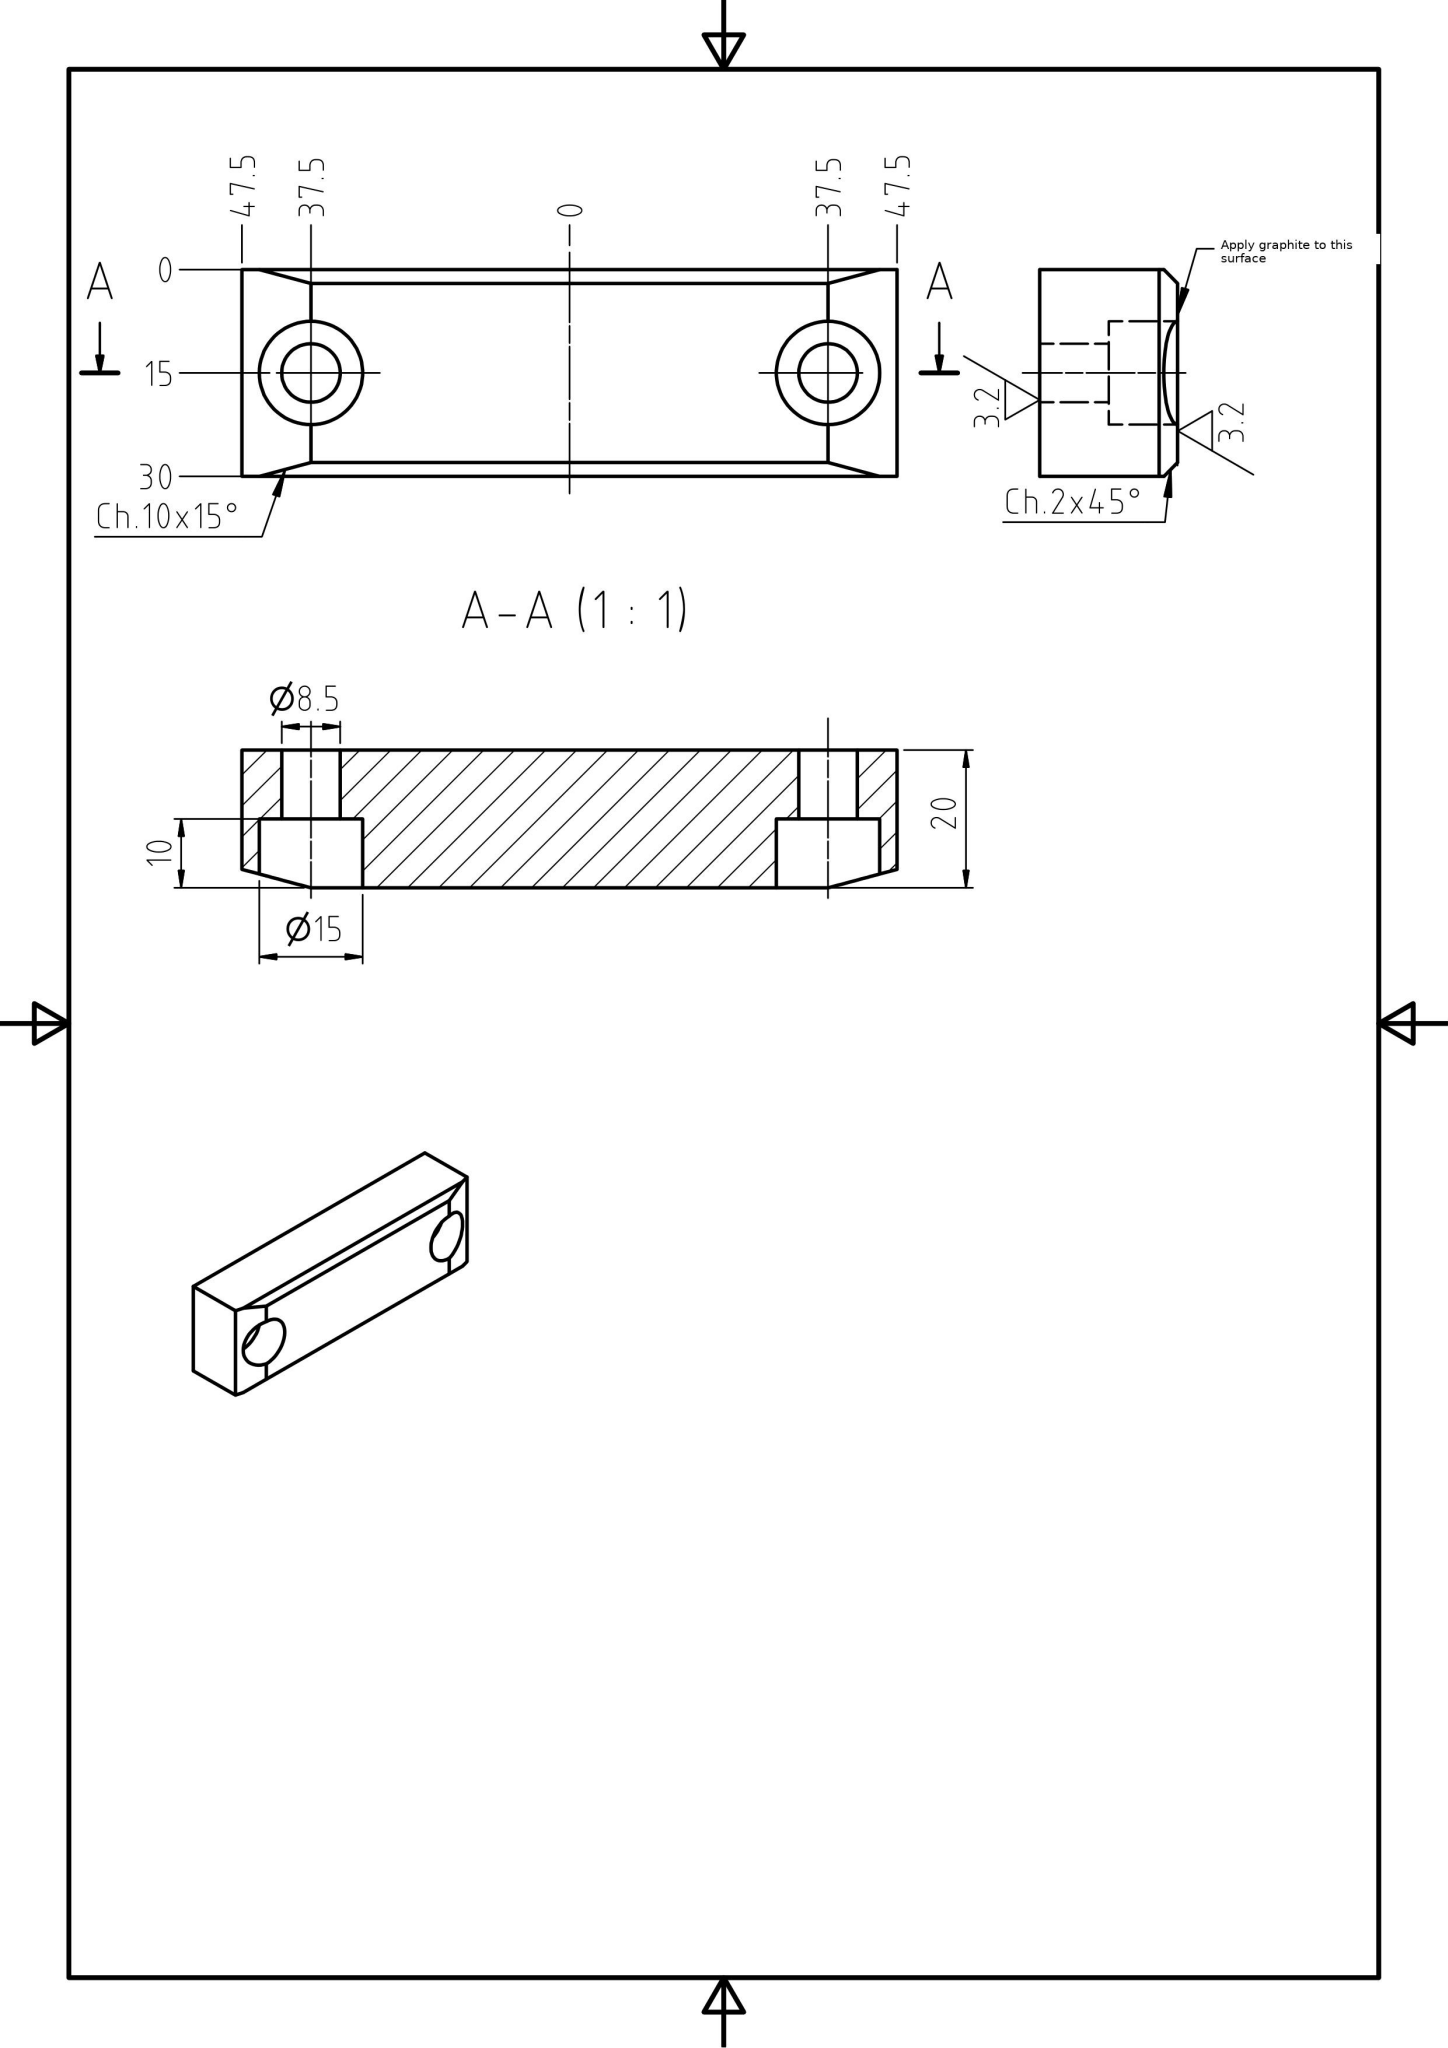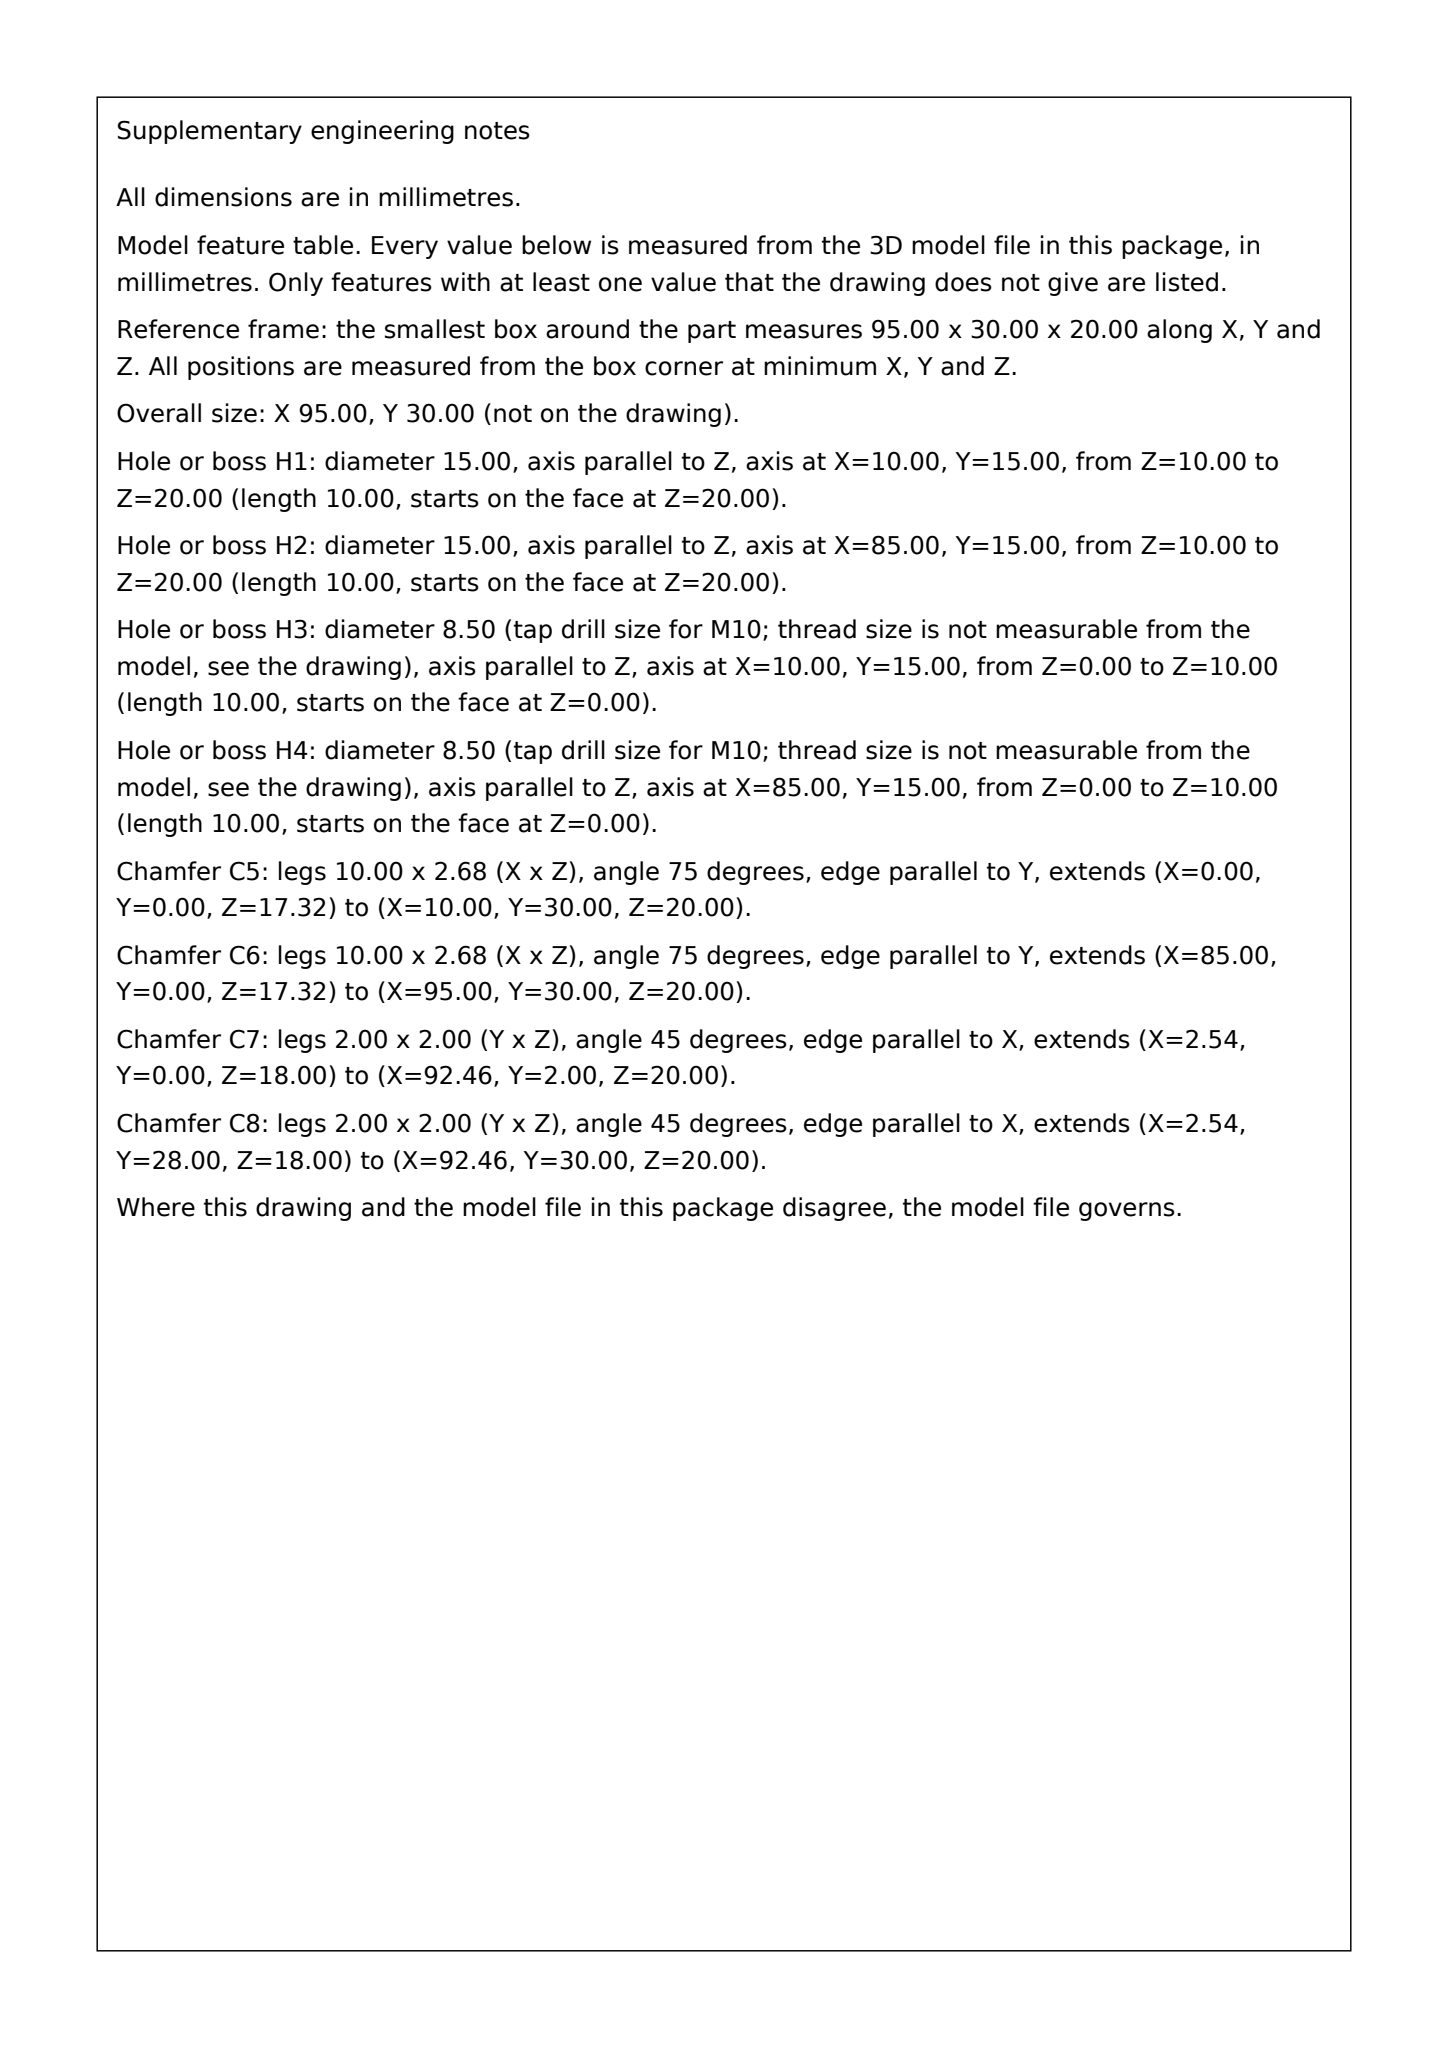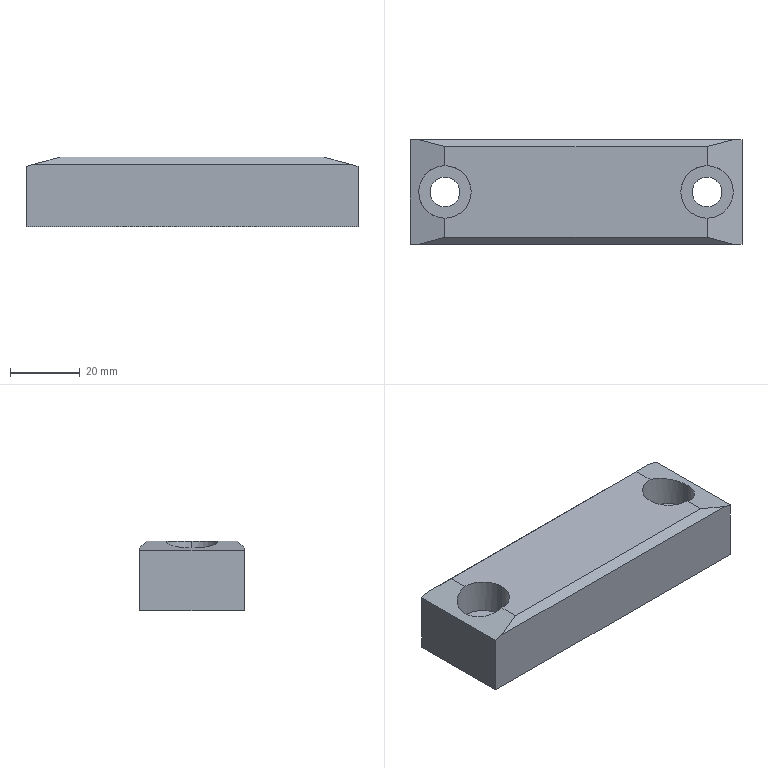Part | SolidWorks | mm | 1 solid | 20 faces | box 95 x 30 x 20 mm | volume 51358 mm3 | plane 12 | cylinder 8 | commonest cylinder face diameters 8.5 x4 15 x4
STEP:
#1=CARTESIAN_POINT('',(33.25,0.,0.));
#2=VERTEX_POINT('',#1);
#3=CARTESIAN_POINT('',(41.75,0.,0.));
#4=VERTEX_POINT('',#3);
#5=CARTESIAN_POINT('',(37.5,0.,0.));
#6=DIRECTION('',(0.,0.,1.));
#7=DIRECTION('',(1.,0.,0.));
#8=AXIS2_PLACEMENT_3D('',#5,#6,#7);
#9=CIRCLE('',#8,4.25);
#10=EDGE_CURVE('',#2,#4,#9,.T.);
#11=ORIENTED_EDGE('',*,*,#10,.F.);
#12=CARTESIAN_POINT('',(33.25,0.,10.));
#13=VERTEX_POINT('',#12);
#14=CARTESIAN_POINT('',(33.25,0.,5.));
#15=DIRECTION('',(0.,0.,1.));
#16=VECTOR('',#15,1000.);
#17=LINE('',#14,#16);
#18=EDGE_CURVE('',#2,#13,#17,.T.);
#19=ORIENTED_EDGE('',*,*,#18,.T.);
#20=CARTESIAN_POINT('',(41.75,0.,10.));
#21=VERTEX_POINT('',#20);
#22=CARTESIAN_POINT('',(37.5,0.,10.));
#23=DIRECTION('',(0.,0.,1.));
#24=DIRECTION('',(1.,0.,0.));
#25=AXIS2_PLACEMENT_3D('',#22,#23,#24);
#26=CIRCLE('',#25,4.25);
#27=EDGE_CURVE('',#13,#21,#26,.T.);
#28=ORIENTED_EDGE('',*,*,#27,.T.);
#29=CARTESIAN_POINT('',(41.75,0.,5.));
#30=DIRECTION('',(0.,0.,1.));
#31=VECTOR('',#30,1000.);
#32=LINE('',#29,#31);
#33=EDGE_CURVE('',#4,#21,#32,.T.);
#34=ORIENTED_EDGE('',*,*,#33,.F.);
#35=EDGE_LOOP('',(#11,#19,#28,#34));
#36=FACE_OUTER_BOUND('',#35,.T.);
#37=CARTESIAN_POINT('',(37.5,0.,5.));
#38=DIRECTION('',(0.,0.,1.));
#39=DIRECTION('',(1.,0.,0.));
#40=AXIS2_PLACEMENT_3D('',#37,#38,#39);
#41=CYLINDRICAL_SURFACE('',#40,4.25);
#42=ADVANCED_FACE('',(#36),#41,.F.);
#43=CARTESIAN_POINT('',(30.,0.,10.));
#44=VERTEX_POINT('',#43);
#45=CARTESIAN_POINT('',(45.,0.,10.));
#46=VERTEX_POINT('',#45);
#47=CARTESIAN_POINT('',(37.5,0.,10.));
#48=DIRECTION('',(0.,0.,1.));
#49=DIRECTION('',(1.,0.,0.));
#50=AXIS2_PLACEMENT_3D('',#47,#48,#49);
#51=CIRCLE('',#50,7.5);
#52=EDGE_CURVE('',#44,#46,#51,.T.);
#53=ORIENTED_EDGE('',*,*,#52,.F.);
#54=CARTESIAN_POINT('',(30.,0.,20.));
#55=VERTEX_POINT('',#54);
#56=CARTESIAN_POINT('',(30.,0.,15.));
#57=DIRECTION('',(0.,0.,1.));
#58=VECTOR('',#57,1000.);
#59=LINE('',#56,#58);
#60=EDGE_CURVE('',#44,#55,#59,.T.);
#61=ORIENTED_EDGE('',*,*,#60,.T.);
#62=CARTESIAN_POINT('',(37.5,-7.5,20.));
#63=VERTEX_POINT('',#62);
#64=CARTESIAN_POINT('',(37.5,0.,20.));
#65=DIRECTION('',(0.,0.,-1.));
#66=DIRECTION('',(1.,0.,0.));
#67=AXIS2_PLACEMENT_3D('',#64,#65,#66);
#68=CIRCLE('',#67,7.5);
#69=EDGE_CURVE('',#63,#55,#68,.T.);
#70=ORIENTED_EDGE('',*,*,#69,.F.);
#71=CARTESIAN_POINT('',(45.,0.,17.99));
#72=VERTEX_POINT('',#71);
#73=CARTESIAN_POINT('',(45.,0.,17.99));
#74=CARTESIAN_POINT('',(45.,-4.393,17.99));
#75=CARTESIAN_POINT('',(41.893,-7.5,18.823));
#76=CARTESIAN_POINT('',(37.5,-7.5,20.));
#77=(BOUNDED_CURVE()B_SPLINE_CURVE(3,(#73,#74,#75,#76),.UNSPECIFIED.,.F.,.F.)B_SPLINE_CURVE_WITH_KNOTS((4,4),(0.,1.571),.UNSPECIFIED.)CURVE()GEOMETRIC_REPRESENTATION_ITEM()RATIONAL_B_SPLINE_CURVE((1.,0.8047,0.8047,1.))REPRESENTATION_ITEM(''));
#78=EDGE_CURVE('',#72,#63,#77,.T.);
#79=ORIENTED_EDGE('',*,*,#78,.F.);
#80=CARTESIAN_POINT('',(45.,0.,15.));
#81=DIRECTION('',(0.,0.,1.));
#82=VECTOR('',#81,1000.);
#83=LINE('',#80,#82);
#84=EDGE_CURVE('',#46,#72,#83,.T.);
#85=ORIENTED_EDGE('',*,*,#84,.F.);
#86=EDGE_LOOP('',(#53,#61,#70,#79,#85));
#87=FACE_OUTER_BOUND('',#86,.T.);
#88=CARTESIAN_POINT('',(37.5,0.,15.));
#89=DIRECTION('',(0.,0.,1.));
#90=DIRECTION('',(1.,0.,0.));
#91=AXIS2_PLACEMENT_3D('',#88,#89,#90);
#92=CYLINDRICAL_SURFACE('',#91,7.5);
#93=ADVANCED_FACE('',(#87),#92,.F.);
#94=CARTESIAN_POINT('',(-41.75,0.,0.));
#95=VERTEX_POINT('',#94);
#96=CARTESIAN_POINT('',(-33.25,0.,0.));
#97=VERTEX_POINT('',#96);
#98=CARTESIAN_POINT('',(-37.5,0.,0.));
#99=DIRECTION('',(0.,0.,1.));
#100=DIRECTION('',(1.,0.,0.));
#101=AXIS2_PLACEMENT_3D('',#98,#99,#100);
#102=CIRCLE('',#101,4.25);
#103=EDGE_CURVE('',#95,#97,#102,.T.);
#104=ORIENTED_EDGE('',*,*,#103,.F.);
#105=CARTESIAN_POINT('',(-41.75,0.,10.));
#106=VERTEX_POINT('',#105);
#107=CARTESIAN_POINT('',(-41.75,0.,5.));
#108=DIRECTION('',(0.,0.,1.));
#109=VECTOR('',#108,1000.);
#110=LINE('',#107,#109);
#111=EDGE_CURVE('',#95,#106,#110,.T.);
#112=ORIENTED_EDGE('',*,*,#111,.T.);
#113=CARTESIAN_POINT('',(-33.25,0.,10.));
#114=VERTEX_POINT('',#113);
#115=CARTESIAN_POINT('',(-37.5,0.,10.));
#116=DIRECTION('',(0.,0.,1.));
#117=DIRECTION('',(1.,0.,0.));
#118=AXIS2_PLACEMENT_3D('',#115,#116,#117);
#119=CIRCLE('',#118,4.25);
#120=EDGE_CURVE('',#106,#114,#119,.T.);
#121=ORIENTED_EDGE('',*,*,#120,.T.);
#122=CARTESIAN_POINT('',(-33.25,0.,5.));
#123=DIRECTION('',(0.,0.,1.));
#124=VECTOR('',#123,1000.);
#125=LINE('',#122,#124);
#126=EDGE_CURVE('',#97,#114,#125,.T.);
#127=ORIENTED_EDGE('',*,*,#126,.F.);
#128=EDGE_LOOP('',(#104,#112,#121,#127));
#129=FACE_OUTER_BOUND('',#128,.T.);
#130=CARTESIAN_POINT('',(-37.5,0.,5.));
#131=DIRECTION('',(0.,0.,1.));
#132=DIRECTION('',(1.,0.,0.));
#133=AXIS2_PLACEMENT_3D('',#130,#131,#132);
#134=CYLINDRICAL_SURFACE('',#133,4.25);
#135=ADVANCED_FACE('',(#129),#134,.F.);
#136=CARTESIAN_POINT('',(-45.,0.,10.));
#137=VERTEX_POINT('',#136);
#138=CARTESIAN_POINT('',(-30.,0.,10.));
#139=VERTEX_POINT('',#138);
#140=CARTESIAN_POINT('',(-37.5,0.,10.));
#141=DIRECTION('',(0.,0.,1.));
#142=DIRECTION('',(1.,0.,0.));
#143=AXIS2_PLACEMENT_3D('',#140,#141,#142);
#144=CIRCLE('',#143,7.5);
#145=EDGE_CURVE('',#137,#139,#144,.T.);
#146=ORIENTED_EDGE('',*,*,#145,.F.);
#147=CARTESIAN_POINT('',(-45.,0.,17.99));
#148=VERTEX_POINT('',#147);
#149=CARTESIAN_POINT('',(-45.,0.,15.));
#150=DIRECTION('',(0.,0.,1.));
#151=VECTOR('',#150,1000.);
#152=LINE('',#149,#151);
#153=EDGE_CURVE('',#137,#148,#152,.T.);
#154=ORIENTED_EDGE('',*,*,#153,.T.);
#155=CARTESIAN_POINT('',(-37.5,-7.5,20.));
#156=VERTEX_POINT('',#155);
#157=CARTESIAN_POINT('',(-37.5,-7.5,20.));
#158=CARTESIAN_POINT('',(-41.893,-7.5,18.823));
#159=CARTESIAN_POINT('',(-45.,-4.393,17.99));
#160=CARTESIAN_POINT('',(-45.,0.,17.99));
#161=(BOUNDED_CURVE()B_SPLINE_CURVE(3,(#157,#158,#159,#160),.UNSPECIFIED.,.F.,.F.)B_SPLINE_CURVE_WITH_KNOTS((4,4),(1.571,3.142),.UNSPECIFIED.)CURVE()GEOMETRIC_REPRESENTATION_ITEM()RATIONAL_B_SPLINE_CURVE((1.,0.8047,0.8047,1.))REPRESENTATION_ITEM(''));
#162=EDGE_CURVE('',#156,#148,#161,.T.);
#163=ORIENTED_EDGE('',*,*,#162,.F.);
#164=CARTESIAN_POINT('',(-30.,0.,20.));
#165=VERTEX_POINT('',#164);
#166=CARTESIAN_POINT('',(-37.5,0.,20.));
#167=DIRECTION('',(0.,0.,-1.));
#168=DIRECTION('',(1.,0.,0.));
#169=AXIS2_PLACEMENT_3D('',#166,#167,#168);
#170=CIRCLE('',#169,7.5);
#171=EDGE_CURVE('',#165,#156,#170,.T.);
#172=ORIENTED_EDGE('',*,*,#171,.F.);
#173=CARTESIAN_POINT('',(-30.,0.,15.));
#174=DIRECTION('',(0.,0.,1.));
#175=VECTOR('',#174,1000.);
#176=LINE('',#173,#175);
#177=EDGE_CURVE('',#139,#165,#176,.T.);
#178=ORIENTED_EDGE('',*,*,#177,.F.);
#179=EDGE_LOOP('',(#146,#154,#163,#172,#178));
#180=FACE_OUTER_BOUND('',#179,.T.);
#181=CARTESIAN_POINT('',(-37.5,0.,15.));
#182=DIRECTION('',(0.,0.,1.));
#183=DIRECTION('',(1.,0.,0.));
#184=AXIS2_PLACEMENT_3D('',#181,#182,#183);
#185=CYLINDRICAL_SURFACE('',#184,7.5);
#186=ADVANCED_FACE('',(#180),#185,.F.);
#187=CARTESIAN_POINT('',(44.964,-15.,18.));
#188=VERTEX_POINT('',#187);
#189=CARTESIAN_POINT('',(37.5,-13.,20.));
#190=VERTEX_POINT('',#189);
#191=CARTESIAN_POINT('',(12.653,-6.342,26.658));
#192=DIRECTION('',(-0.9351,0.2506,0.2506));
#193=VECTOR('',#192,1000.);
#194=LINE('',#191,#193);
#195=EDGE_CURVE('',#188,#190,#194,.T.);
#196=ORIENTED_EDGE('',*,*,#195,.T.);
#197=CARTESIAN_POINT('',(-37.5,-13.,20.));
#198=VERTEX_POINT('',#197);
#199=CARTESIAN_POINT('',(-23.75,-13.,20.));
#200=DIRECTION('',(-1.,0.,0.));
#201=VECTOR('',#200,1000.);
#202=LINE('',#199,#201);
#203=EDGE_CURVE('',#190,#198,#202,.T.);
#204=ORIENTED_EDGE('',*,*,#203,.T.);
#205=CARTESIAN_POINT('',(-44.964,-15.,18.));
#206=VERTEX_POINT('',#205);
#207=CARTESIAN_POINT('',(-31.664,-11.436,21.564));
#208=DIRECTION('',(-0.9351,-0.2506,-0.2506));
#209=VECTOR('',#208,1000.);
#210=LINE('',#207,#209);
#211=EDGE_CURVE('',#198,#206,#210,.T.);
#212=ORIENTED_EDGE('',*,*,#211,.T.);
#213=CARTESIAN_POINT('',(-23.75,-15.,18.));
#214=DIRECTION('',(1.,0.,0.));
#215=VECTOR('',#214,1000.);
#216=LINE('',#213,#215);
#217=EDGE_CURVE('',#206,#188,#216,.T.);
#218=ORIENTED_EDGE('',*,*,#217,.T.);
#219=EDGE_LOOP('',(#196,#204,#212,#218));
#220=FACE_OUTER_BOUND('',#219,.T.);
#221=CARTESIAN_POINT('',(-23.75,-14.,19.));
#222=DIRECTION('',(0.,-0.7071,0.7071));
#223=DIRECTION('',(-1.,0.,0.));
#224=AXIS2_PLACEMENT_3D('',#221,#222,#223);
#225=PLANE('',#224);
#226=ADVANCED_FACE('',(#220),#225,.T.);
#227=ORIENTED_EDGE('',*,*,#211,.F.);
#228=CARTESIAN_POINT('',(-37.5,7.5,20.));
#229=DIRECTION('',(0.,1.,0.));
#230=VECTOR('',#229,1000.);
#231=LINE('',#228,#230);
#232=EDGE_CURVE('',#198,#156,#231,.T.);
#233=ORIENTED_EDGE('',*,*,#232,.T.);
#234=ORIENTED_EDGE('',*,*,#162,.T.);
#235=CARTESIAN_POINT('',(-37.5,7.5,20.));
#236=VERTEX_POINT('',#235);
#237=CARTESIAN_POINT('',(-45.,0.,17.99));
#238=CARTESIAN_POINT('',(-45.,4.393,17.99));
#239=CARTESIAN_POINT('',(-41.893,7.5,18.823));
#240=CARTESIAN_POINT('',(-37.5,7.5,20.));
#241=(BOUNDED_CURVE()B_SPLINE_CURVE(3,(#237,#238,#239,#240),.UNSPECIFIED.,.F.,.F.)B_SPLINE_CURVE_WITH_KNOTS((4,4),(3.142,4.712),.UNSPECIFIED.)CURVE()GEOMETRIC_REPRESENTATION_ITEM()RATIONAL_B_SPLINE_CURVE((1.,0.8047,0.8047,1.))REPRESENTATION_ITEM(''));
#242=EDGE_CURVE('',#148,#236,#241,.T.);
#243=ORIENTED_EDGE('',*,*,#242,.T.);
#244=CARTESIAN_POINT('',(-37.5,13.,20.));
#245=VERTEX_POINT('',#244);
#246=CARTESIAN_POINT('',(-37.5,7.5,20.));
#247=DIRECTION('',(0.,1.,0.));
#248=VECTOR('',#247,1000.);
#249=LINE('',#246,#248);
#250=EDGE_CURVE('',#236,#245,#249,.T.);
#251=ORIENTED_EDGE('',*,*,#250,.T.);
#252=CARTESIAN_POINT('',(-44.964,15.,18.));
#253=VERTEX_POINT('',#252);
#254=CARTESIAN_POINT('',(-12.653,6.342,26.658));
#255=DIRECTION('',(0.9351,-0.2506,0.2506));
#256=VECTOR('',#255,1000.);
#257=LINE('',#254,#256);
#258=EDGE_CURVE('',#253,#245,#257,.T.);
#259=ORIENTED_EDGE('',*,*,#258,.F.);
#260=CARTESIAN_POINT('',(-47.5,15.,17.321));
#261=VERTEX_POINT('',#260);
#262=CARTESIAN_POINT('',(-2.847,15.,29.285));
#263=DIRECTION('',(-0.9659,0.,-0.2588));
#264=VECTOR('',#263,1000.);
#265=LINE('',#262,#264);
#266=EDGE_CURVE('',#253,#261,#265,.T.);
#267=ORIENTED_EDGE('',*,*,#266,.T.);
#268=CARTESIAN_POINT('',(-47.5,-15.,17.321));
#269=VERTEX_POINT('',#268);
#270=CARTESIAN_POINT('',(-47.5,7.5,17.321));
#271=DIRECTION('',(0.,-1.,0.));
#272=VECTOR('',#271,1000.);
#273=LINE('',#270,#272);
#274=EDGE_CURVE('',#261,#269,#273,.T.);
#275=ORIENTED_EDGE('',*,*,#274,.T.);
#276=CARTESIAN_POINT('',(-47.165,-15.,17.41));
#277=DIRECTION('',(0.9659,0.,0.2588));
#278=VECTOR('',#277,1000.);
#279=LINE('',#276,#278);
#280=EDGE_CURVE('',#269,#206,#279,.T.);
#281=ORIENTED_EDGE('',*,*,#280,.T.);
#282=EDGE_LOOP('',(#227,#233,#234,#243,#251,#259,#267,#275,#281));
#283=FACE_OUTER_BOUND('',#282,.T.);
#284=CARTESIAN_POINT('',(-42.5,7.5,18.66));
#285=DIRECTION('',(-0.2588,0.,0.9659));
#286=DIRECTION('',(0.,1.,0.));
#287=AXIS2_PLACEMENT_3D('',#284,#285,#286);
#288=PLANE('',#287);
#289=ADVANCED_FACE('',(#283),#288,.T.);
#290=ORIENTED_EDGE('',*,*,#203,.F.);
#291=CARTESIAN_POINT('',(37.5,-7.5,20.));
#292=DIRECTION('',(0.,-1.,0.));
#293=VECTOR('',#292,1000.);
#294=LINE('',#291,#293);
#295=EDGE_CURVE('',#63,#190,#294,.T.);
#296=ORIENTED_EDGE('',*,*,#295,.F.);
#297=ORIENTED_EDGE('',*,*,#69,.T.);
#298=CARTESIAN_POINT('',(37.5,7.5,20.));
#299=VERTEX_POINT('',#298);
#300=CARTESIAN_POINT('',(37.5,0.,20.));
#301=DIRECTION('',(0.,0.,-1.));
#302=DIRECTION('',(1.,0.,0.));
#303=AXIS2_PLACEMENT_3D('',#300,#301,#302);
#304=CIRCLE('',#303,7.5);
#305=EDGE_CURVE('',#55,#299,#304,.T.);
#306=ORIENTED_EDGE('',*,*,#305,.T.);
#307=CARTESIAN_POINT('',(37.5,13.,20.));
#308=VERTEX_POINT('',#307);
#309=CARTESIAN_POINT('',(37.5,-7.5,20.));
#310=DIRECTION('',(0.,-1.,0.));
#311=VECTOR('',#310,1000.);
#312=LINE('',#309,#311);
#313=EDGE_CURVE('',#308,#299,#312,.T.);
#314=ORIENTED_EDGE('',*,*,#313,.F.);
#315=CARTESIAN_POINT('',(23.75,13.,20.));
#316=DIRECTION('',(1.,0.,0.));
#317=VECTOR('',#316,1000.);
#318=LINE('',#315,#317);
#319=EDGE_CURVE('',#245,#308,#318,.T.);
#320=ORIENTED_EDGE('',*,*,#319,.F.);
#321=ORIENTED_EDGE('',*,*,#250,.F.);
#322=CARTESIAN_POINT('',(-37.5,0.,20.));
#323=DIRECTION('',(0.,0.,-1.));
#324=DIRECTION('',(1.,0.,0.));
#325=AXIS2_PLACEMENT_3D('',#322,#323,#324);
#326=CIRCLE('',#325,7.5);
#327=EDGE_CURVE('',#236,#165,#326,.T.);
#328=ORIENTED_EDGE('',*,*,#327,.T.);
#329=ORIENTED_EDGE('',*,*,#171,.T.);
#330=ORIENTED_EDGE('',*,*,#232,.F.);
#331=EDGE_LOOP('',(#290,#296,#297,#306,#314,#320,#321,#328,#329,#330));
#332=FACE_OUTER_BOUND('',#331,.T.);
#333=CARTESIAN_POINT('',(0.,0.,20.));
#334=DIRECTION('',(0.,0.,1.));
#335=DIRECTION('',(1.,0.,0.));
#336=AXIS2_PLACEMENT_3D('',#333,#334,#335);
#337=PLANE('',#336);
#338=ADVANCED_FACE('',(#332),#337,.T.);
#339=ORIENTED_EDGE('',*,*,#258,.T.);
#340=ORIENTED_EDGE('',*,*,#319,.T.);
#341=CARTESIAN_POINT('',(44.964,15.,18.));
#342=VERTEX_POINT('',#341);
#343=CARTESIAN_POINT('',(31.664,11.436,21.564));
#344=DIRECTION('',(0.9351,0.2506,-0.2506));
#345=VECTOR('',#344,1000.);
#346=LINE('',#343,#345);
#347=EDGE_CURVE('',#308,#342,#346,.T.);
#348=ORIENTED_EDGE('',*,*,#347,.T.);
#349=CARTESIAN_POINT('',(23.75,15.,18.));
#350=DIRECTION('',(-1.,0.,0.));
#351=VECTOR('',#350,1000.);
#352=LINE('',#349,#351);
#353=EDGE_CURVE('',#342,#253,#352,.T.);
#354=ORIENTED_EDGE('',*,*,#353,.T.);
#355=EDGE_LOOP('',(#339,#340,#348,#354));
#356=FACE_OUTER_BOUND('',#355,.T.);
#357=CARTESIAN_POINT('',(23.75,14.,19.));
#358=DIRECTION('',(0.,0.7071,0.7071));
#359=DIRECTION('',(1.,0.,0.));
#360=AXIS2_PLACEMENT_3D('',#357,#358,#359);
#361=PLANE('',#360);
#362=ADVANCED_FACE('',(#356),#361,.T.);
#363=ORIENTED_EDGE('',*,*,#274,.F.);
#364=CARTESIAN_POINT('',(-47.5,15.,0.));
#365=VERTEX_POINT('',#364);
#366=CARTESIAN_POINT('',(-47.5,15.,0.));
#367=DIRECTION('',(0.,0.,1.));
#368=VECTOR('',#367,1000.);
#369=LINE('',#366,#368);
#370=EDGE_CURVE('',#365,#261,#369,.T.);
#371=ORIENTED_EDGE('',*,*,#370,.F.);
#372=CARTESIAN_POINT('',(-47.5,-15.,0.));
#373=VERTEX_POINT('',#372);
#374=CARTESIAN_POINT('',(-47.5,-15.,0.));
#375=DIRECTION('',(0.,1.,0.));
#376=VECTOR('',#375,1000.);
#377=LINE('',#374,#376);
#378=EDGE_CURVE('',#373,#365,#377,.T.);
#379=ORIENTED_EDGE('',*,*,#378,.F.);
#380=CARTESIAN_POINT('',(-47.5,-15.,0.));
#381=DIRECTION('',(0.,0.,1.));
#382=VECTOR('',#381,1000.);
#383=LINE('',#380,#382);
#384=EDGE_CURVE('',#373,#269,#383,.T.);
#385=ORIENTED_EDGE('',*,*,#384,.T.);
#386=EDGE_LOOP('',(#363,#371,#379,#385));
#387=FACE_OUTER_BOUND('',#386,.T.);
#388=CARTESIAN_POINT('',(-47.5,15.,0.));
#389=DIRECTION('',(-1.,0.,0.));
#390=DIRECTION('',(0.,0.,1.));
#391=AXIS2_PLACEMENT_3D('',#388,#389,#390);
#392=PLANE('',#391);
#393=ADVANCED_FACE('',(#387),#392,.T.);
#394=ORIENTED_EDGE('',*,*,#353,.F.);
#395=CARTESIAN_POINT('',(47.5,15.,17.321));
#396=VERTEX_POINT('',#395);
#397=CARTESIAN_POINT('',(47.165,15.,17.41));
#398=DIRECTION('',(-0.9659,0.,0.2588));
#399=VECTOR('',#398,1000.);
#400=LINE('',#397,#399);
#401=EDGE_CURVE('',#396,#342,#400,.T.);
#402=ORIENTED_EDGE('',*,*,#401,.F.);
#403=CARTESIAN_POINT('',(47.5,15.,0.));
#404=VERTEX_POINT('',#403);
#405=CARTESIAN_POINT('',(47.5,15.,0.));
#406=DIRECTION('',(0.,0.,1.));
#407=VECTOR('',#406,1000.);
#408=LINE('',#405,#407);
#409=EDGE_CURVE('',#404,#396,#408,.T.);
#410=ORIENTED_EDGE('',*,*,#409,.F.);
#411=CARTESIAN_POINT('',(-47.5,15.,0.));
#412=DIRECTION('',(1.,0.,0.));
#413=VECTOR('',#412,1000.);
#414=LINE('',#411,#413);
#415=EDGE_CURVE('',#365,#404,#414,.T.);
#416=ORIENTED_EDGE('',*,*,#415,.F.);
#417=ORIENTED_EDGE('',*,*,#370,.T.);
#418=ORIENTED_EDGE('',*,*,#266,.F.);
#419=EDGE_LOOP('',(#394,#402,#410,#416,#417,#418));
#420=FACE_OUTER_BOUND('',#419,.T.);
#421=CARTESIAN_POINT('',(47.5,15.,0.));
#422=DIRECTION('',(0.,1.,0.));
#423=DIRECTION('',(1.,0.,0.));
#424=AXIS2_PLACEMENT_3D('',#421,#422,#423);
#425=PLANE('',#424);
#426=ADVANCED_FACE('',(#420),#425,.T.);
#427=ORIENTED_EDGE('',*,*,#195,.F.);
#428=CARTESIAN_POINT('',(47.5,-15.,17.321));
#429=VERTEX_POINT('',#428);
#430=CARTESIAN_POINT('',(2.847,-15.,29.285));
#431=DIRECTION('',(0.9659,0.,-0.2588));
#432=VECTOR('',#431,1000.);
#433=LINE('',#430,#432);
#434=EDGE_CURVE('',#188,#429,#433,.T.);
#435=ORIENTED_EDGE('',*,*,#434,.T.);
#436=CARTESIAN_POINT('',(47.5,-7.5,17.321));
#437=DIRECTION('',(0.,1.,0.));
#438=VECTOR('',#437,1000.);
#439=LINE('',#436,#438);
#440=EDGE_CURVE('',#429,#396,#439,.T.);
#441=ORIENTED_EDGE('',*,*,#440,.T.);
#442=ORIENTED_EDGE('',*,*,#401,.T.);
#443=ORIENTED_EDGE('',*,*,#347,.F.);
#444=ORIENTED_EDGE('',*,*,#313,.T.);
#445=CARTESIAN_POINT('',(37.5,7.5,20.));
#446=CARTESIAN_POINT('',(41.893,7.5,18.823));
#447=CARTESIAN_POINT('',(45.,4.393,17.99));
#448=CARTESIAN_POINT('',(45.,0.,17.99));
#449=(BOUNDED_CURVE()B_SPLINE_CURVE(3,(#445,#446,#447,#448),.UNSPECIFIED.,.F.,.T.)B_SPLINE_CURVE_WITH_KNOTS((4,4),(4.712,6.283),.UNSPECIFIED.)CURVE()GEOMETRIC_REPRESENTATION_ITEM()RATIONAL_B_SPLINE_CURVE((1.,0.8047,0.8047,1.))REPRESENTATION_ITEM(''));
#450=EDGE_CURVE('',#299,#72,#449,.T.);
#451=ORIENTED_EDGE('',*,*,#450,.T.);
#452=ORIENTED_EDGE('',*,*,#78,.T.);
#453=ORIENTED_EDGE('',*,*,#295,.T.);
#454=EDGE_LOOP('',(#427,#435,#441,#442,#443,#444,#451,#452,#453));
#455=FACE_OUTER_BOUND('',#454,.T.);
#456=CARTESIAN_POINT('',(42.5,-7.5,18.66));
#457=DIRECTION('',(0.2588,0.,0.9659));
#458=DIRECTION('',(0.,-1.,0.));
#459=AXIS2_PLACEMENT_3D('',#456,#457,#458);
#460=PLANE('',#459);
#461=ADVANCED_FACE('',(#455),#460,.T.);
#462=ORIENTED_EDGE('',*,*,#440,.F.);
#463=CARTESIAN_POINT('',(47.5,-15.,0.));
#464=VERTEX_POINT('',#463);
#465=CARTESIAN_POINT('',(47.5,-15.,0.));
#466=DIRECTION('',(0.,0.,1.));
#467=VECTOR('',#466,1000.);
#468=LINE('',#465,#467);
#469=EDGE_CURVE('',#464,#429,#468,.T.);
#470=ORIENTED_EDGE('',*,*,#469,.F.);
#471=CARTESIAN_POINT('',(47.5,15.,0.));
#472=DIRECTION('',(0.,-1.,0.));
#473=VECTOR('',#472,1000.);
#474=LINE('',#471,#473);
#475=EDGE_CURVE('',#404,#464,#474,.T.);
#476=ORIENTED_EDGE('',*,*,#475,.F.);
#477=ORIENTED_EDGE('',*,*,#409,.T.);
#478=EDGE_LOOP('',(#462,#470,#476,#477));
#479=FACE_OUTER_BOUND('',#478,.T.);
#480=CARTESIAN_POINT('',(47.5,-15.,0.));
#481=DIRECTION('',(1.,0.,0.));
#482=DIRECTION('',(0.,1.,0.));
#483=AXIS2_PLACEMENT_3D('',#480,#481,#482);
#484=PLANE('',#483);
#485=ADVANCED_FACE('',(#479),#484,.T.);
#486=CARTESIAN_POINT('',(-37.5,0.,10.));
#487=DIRECTION('',(0.,0.,1.));
#488=DIRECTION('',(1.,0.,0.));
#489=AXIS2_PLACEMENT_3D('',#486,#487,#488);
#490=CIRCLE('',#489,7.5);
#491=EDGE_CURVE('',#139,#137,#490,.T.);
#492=ORIENTED_EDGE('',*,*,#491,.T.);
#493=ORIENTED_EDGE('',*,*,#145,.T.);
#494=EDGE_LOOP('',(#492,#493));
#495=FACE_OUTER_BOUND('',#494,.T.);
#496=CARTESIAN_POINT('',(-37.5,0.,10.));
#497=DIRECTION('',(0.,0.,1.));
#498=DIRECTION('',(1.,0.,0.));
#499=AXIS2_PLACEMENT_3D('',#496,#497,#498);
#500=CIRCLE('',#499,4.25);
#501=EDGE_CURVE('',#114,#106,#500,.T.);
#502=ORIENTED_EDGE('',*,*,#501,.F.);
#503=ORIENTED_EDGE('',*,*,#120,.F.);
#504=EDGE_LOOP('',(#502,#503));
#505=FACE_BOUND('',#504,.T.);
#506=CARTESIAN_POINT('',(-37.5,0.,10.));
#507=DIRECTION('',(0.,0.,1.));
#508=DIRECTION('',(1.,0.,0.));
#509=AXIS2_PLACEMENT_3D('',#506,#507,#508);
#510=PLANE('',#509);
#511=ADVANCED_FACE('',(#495,#505),#510,.T.);
#512=ORIENTED_EDGE('',*,*,#153,.F.);
#513=ORIENTED_EDGE('',*,*,#491,.F.);
#514=ORIENTED_EDGE('',*,*,#177,.T.);
#515=ORIENTED_EDGE('',*,*,#327,.F.);
#516=ORIENTED_EDGE('',*,*,#242,.F.);
#517=EDGE_LOOP('',(#512,#513,#514,#515,#516));
#518=FACE_OUTER_BOUND('',#517,.T.);
#519=CARTESIAN_POINT('',(-37.5,0.,15.));
#520=DIRECTION('',(0.,0.,1.));
#521=DIRECTION('',(1.,0.,0.));
#522=AXIS2_PLACEMENT_3D('',#519,#520,#521);
#523=CYLINDRICAL_SURFACE('',#522,7.5);
#524=ADVANCED_FACE('',(#518),#523,.F.);
#525=ORIENTED_EDGE('',*,*,#111,.F.);
#526=CARTESIAN_POINT('',(-37.5,0.,0.));
#527=DIRECTION('',(0.,0.,1.));
#528=DIRECTION('',(1.,0.,0.));
#529=AXIS2_PLACEMENT_3D('',#526,#527,#528);
#530=CIRCLE('',#529,4.25);
#531=EDGE_CURVE('',#97,#95,#530,.T.);
#532=ORIENTED_EDGE('',*,*,#531,.F.);
#533=ORIENTED_EDGE('',*,*,#126,.T.);
#534=ORIENTED_EDGE('',*,*,#501,.T.);
#535=EDGE_LOOP('',(#525,#532,#533,#534));
#536=FACE_OUTER_BOUND('',#535,.T.);
#537=CARTESIAN_POINT('',(-37.5,0.,5.));
#538=DIRECTION('',(0.,0.,1.));
#539=DIRECTION('',(1.,0.,0.));
#540=AXIS2_PLACEMENT_3D('',#537,#538,#539);
#541=CYLINDRICAL_SURFACE('',#540,4.25);
#542=ADVANCED_FACE('',(#536),#541,.F.);
#543=CARTESIAN_POINT('',(37.5,0.,10.));
#544=DIRECTION('',(0.,0.,1.));
#545=DIRECTION('',(1.,0.,0.));
#546=AXIS2_PLACEMENT_3D('',#543,#544,#545);
#547=CIRCLE('',#546,7.5);
#548=EDGE_CURVE('',#46,#44,#547,.T.);
#549=ORIENTED_EDGE('',*,*,#548,.T.);
#550=ORIENTED_EDGE('',*,*,#52,.T.);
#551=EDGE_LOOP('',(#549,#550));
#552=FACE_OUTER_BOUND('',#551,.T.);
#553=CARTESIAN_POINT('',(37.5,0.,10.));
#554=DIRECTION('',(0.,0.,1.));
#555=DIRECTION('',(1.,0.,0.));
#556=AXIS2_PLACEMENT_3D('',#553,#554,#555);
#557=CIRCLE('',#556,4.25);
#558=EDGE_CURVE('',#21,#13,#557,.T.);
#559=ORIENTED_EDGE('',*,*,#558,.F.);
#560=ORIENTED_EDGE('',*,*,#27,.F.);
#561=EDGE_LOOP('',(#559,#560));
#562=FACE_BOUND('',#561,.T.);
#563=CARTESIAN_POINT('',(37.5,0.,10.));
#564=DIRECTION('',(0.,0.,1.));
#565=DIRECTION('',(1.,0.,0.));
#566=AXIS2_PLACEMENT_3D('',#563,#564,#565);
#567=PLANE('',#566);
#568=ADVANCED_FACE('',(#552,#562),#567,.T.);
#569=ORIENTED_EDGE('',*,*,#60,.F.);
#570=ORIENTED_EDGE('',*,*,#548,.F.);
#571=ORIENTED_EDGE('',*,*,#84,.T.);
#572=ORIENTED_EDGE('',*,*,#450,.F.);
#573=ORIENTED_EDGE('',*,*,#305,.F.);
#574=EDGE_LOOP('',(#569,#570,#571,#572,#573));
#575=FACE_OUTER_BOUND('',#574,.T.);
#576=CARTESIAN_POINT('',(37.5,0.,15.));
#577=DIRECTION('',(0.,0.,1.));
#578=DIRECTION('',(1.,0.,0.));
#579=AXIS2_PLACEMENT_3D('',#576,#577,#578);
#580=CYLINDRICAL_SURFACE('',#579,7.5);
#581=ADVANCED_FACE('',(#575),#580,.F.);
#582=ORIENTED_EDGE('',*,*,#18,.F.);
#583=CARTESIAN_POINT('',(37.5,0.,0.));
#584=DIRECTION('',(0.,0.,1.));
#585=DIRECTION('',(1.,0.,0.));
#586=AXIS2_PLACEMENT_3D('',#583,#584,#585);
#587=CIRCLE('',#586,4.25);
#588=EDGE_CURVE('',#4,#2,#587,.T.);
#589=ORIENTED_EDGE('',*,*,#588,.F.);
#590=ORIENTED_EDGE('',*,*,#33,.T.);
#591=ORIENTED_EDGE('',*,*,#558,.T.);
#592=EDGE_LOOP('',(#582,#589,#590,#591));
#593=FACE_OUTER_BOUND('',#592,.T.);
#594=CARTESIAN_POINT('',(37.5,0.,5.));
#595=DIRECTION('',(0.,0.,1.));
#596=DIRECTION('',(1.,0.,0.));
#597=AXIS2_PLACEMENT_3D('',#594,#595,#596);
#598=CYLINDRICAL_SURFACE('',#597,4.25);
#599=ADVANCED_FACE('',(#593),#598,.F.);
#600=ORIENTED_EDGE('',*,*,#217,.F.);
#601=ORIENTED_EDGE('',*,*,#280,.F.);
#602=ORIENTED_EDGE('',*,*,#384,.F.);
#603=CARTESIAN_POINT('',(47.5,-15.,0.));
#604=DIRECTION('',(-1.,0.,0.));
#605=VECTOR('',#604,1000.);
#606=LINE('',#603,#605);
#607=EDGE_CURVE('',#464,#373,#606,.T.);
#608=ORIENTED_EDGE('',*,*,#607,.F.);
#609=ORIENTED_EDGE('',*,*,#469,.T.);
#610=ORIENTED_EDGE('',*,*,#434,.F.);
#611=EDGE_LOOP('',(#600,#601,#602,#608,#609,#610));
#612=FACE_OUTER_BOUND('',#611,.T.);
#613=CARTESIAN_POINT('',(-47.5,-15.,0.));
#614=DIRECTION('',(0.,-1.,0.));
#615=DIRECTION('',(0.,0.,-1.));
#616=AXIS2_PLACEMENT_3D('',#613,#614,#615);
#617=PLANE('',#616);
#618=ADVANCED_FACE('',(#612),#617,.T.);
#619=ORIENTED_EDGE('',*,*,#415,.T.);
#620=ORIENTED_EDGE('',*,*,#475,.T.);
#621=ORIENTED_EDGE('',*,*,#607,.T.);
#622=ORIENTED_EDGE('',*,*,#378,.T.);
#623=EDGE_LOOP('',(#619,#620,#621,#622));
#624=FACE_OUTER_BOUND('',#623,.T.);
#625=ORIENTED_EDGE('',*,*,#531,.T.);
#626=ORIENTED_EDGE('',*,*,#103,.T.);
#627=EDGE_LOOP('',(#625,#626));
#628=FACE_BOUND('',#627,.T.);
#629=ORIENTED_EDGE('',*,*,#588,.T.);
#630=ORIENTED_EDGE('',*,*,#10,.T.);
#631=EDGE_LOOP('',(#629,#630));
#632=FACE_BOUND('',#631,.T.);
#633=CARTESIAN_POINT('',(0.,0.,0.));
#634=DIRECTION('',(0.,0.,1.));
#635=DIRECTION('',(1.,0.,0.));
#636=AXIS2_PLACEMENT_3D('',#633,#634,#635);
#637=PLANE('',#636);
#638=ADVANCED_FACE('',(#624,#628,#632),#637,.F.);
#639=CLOSED_SHELL('',(#42,#93,#135,#186,#226,#289,#338,#362,#393,#426,#461,#485,#511,#524,#542,#568,#581,#599,#618,#638));
#640=MANIFOLD_SOLID_BREP('',#639);
#641=CARTESIAN_POINT('',(0.,0.,0.));
#642=DIRECTION('',(0.,0.,1.));
#643=DIRECTION('',(1.,0.,0.));
#644=AXIS2_PLACEMENT_3D('',#641,#642,#643);
#645=(LENGTH_UNIT()NAMED_UNIT(*)SI_UNIT(.MILLI.,.METRE.));
#646=UNCERTAINTY_MEASURE_WITH_UNIT(LENGTH_MEASURE(0.00001),#645,'','');
#647=(NAMED_UNIT(*)PLANE_ANGLE_UNIT()SI_UNIT($,.RADIAN.));
#648=(NAMED_UNIT(*)SI_UNIT($,.STERADIAN.)SOLID_ANGLE_UNIT());
#649=(GEOMETRIC_REPRESENTATION_CONTEXT(3)GLOBAL_UNCERTAINTY_ASSIGNED_CONTEXT((#646))GLOBAL_UNIT_ASSIGNED_CONTEXT((#645,#647,#648))REPRESENTATION_CONTEXT('',''));
#650=ADVANCED_BREP_SHAPE_REPRESENTATION('',(#640,#644),#649);